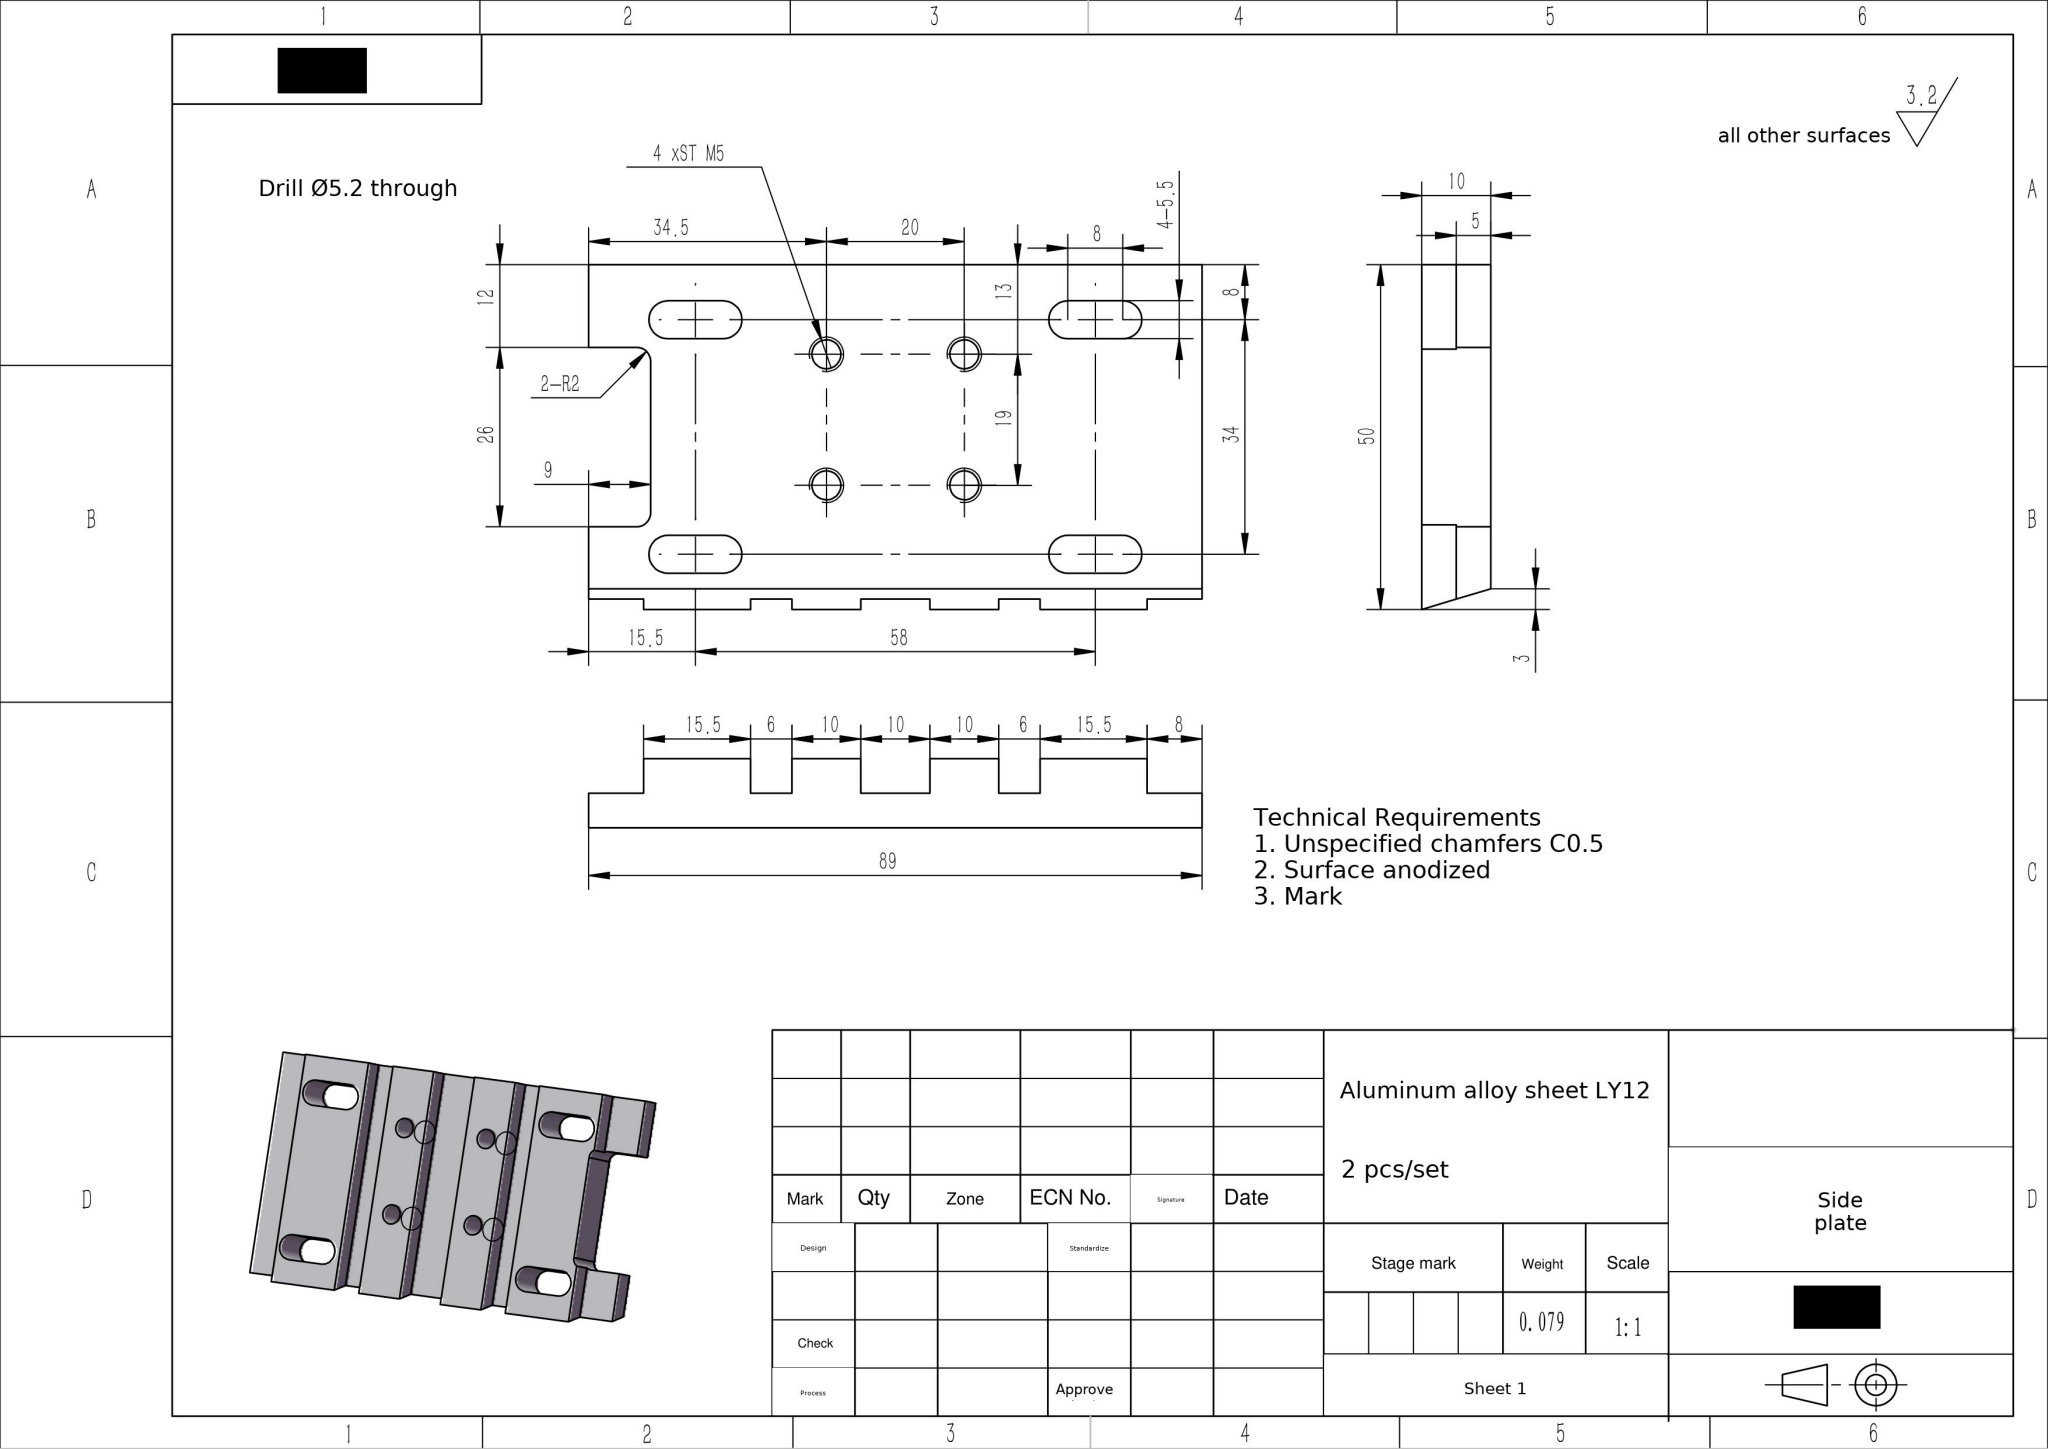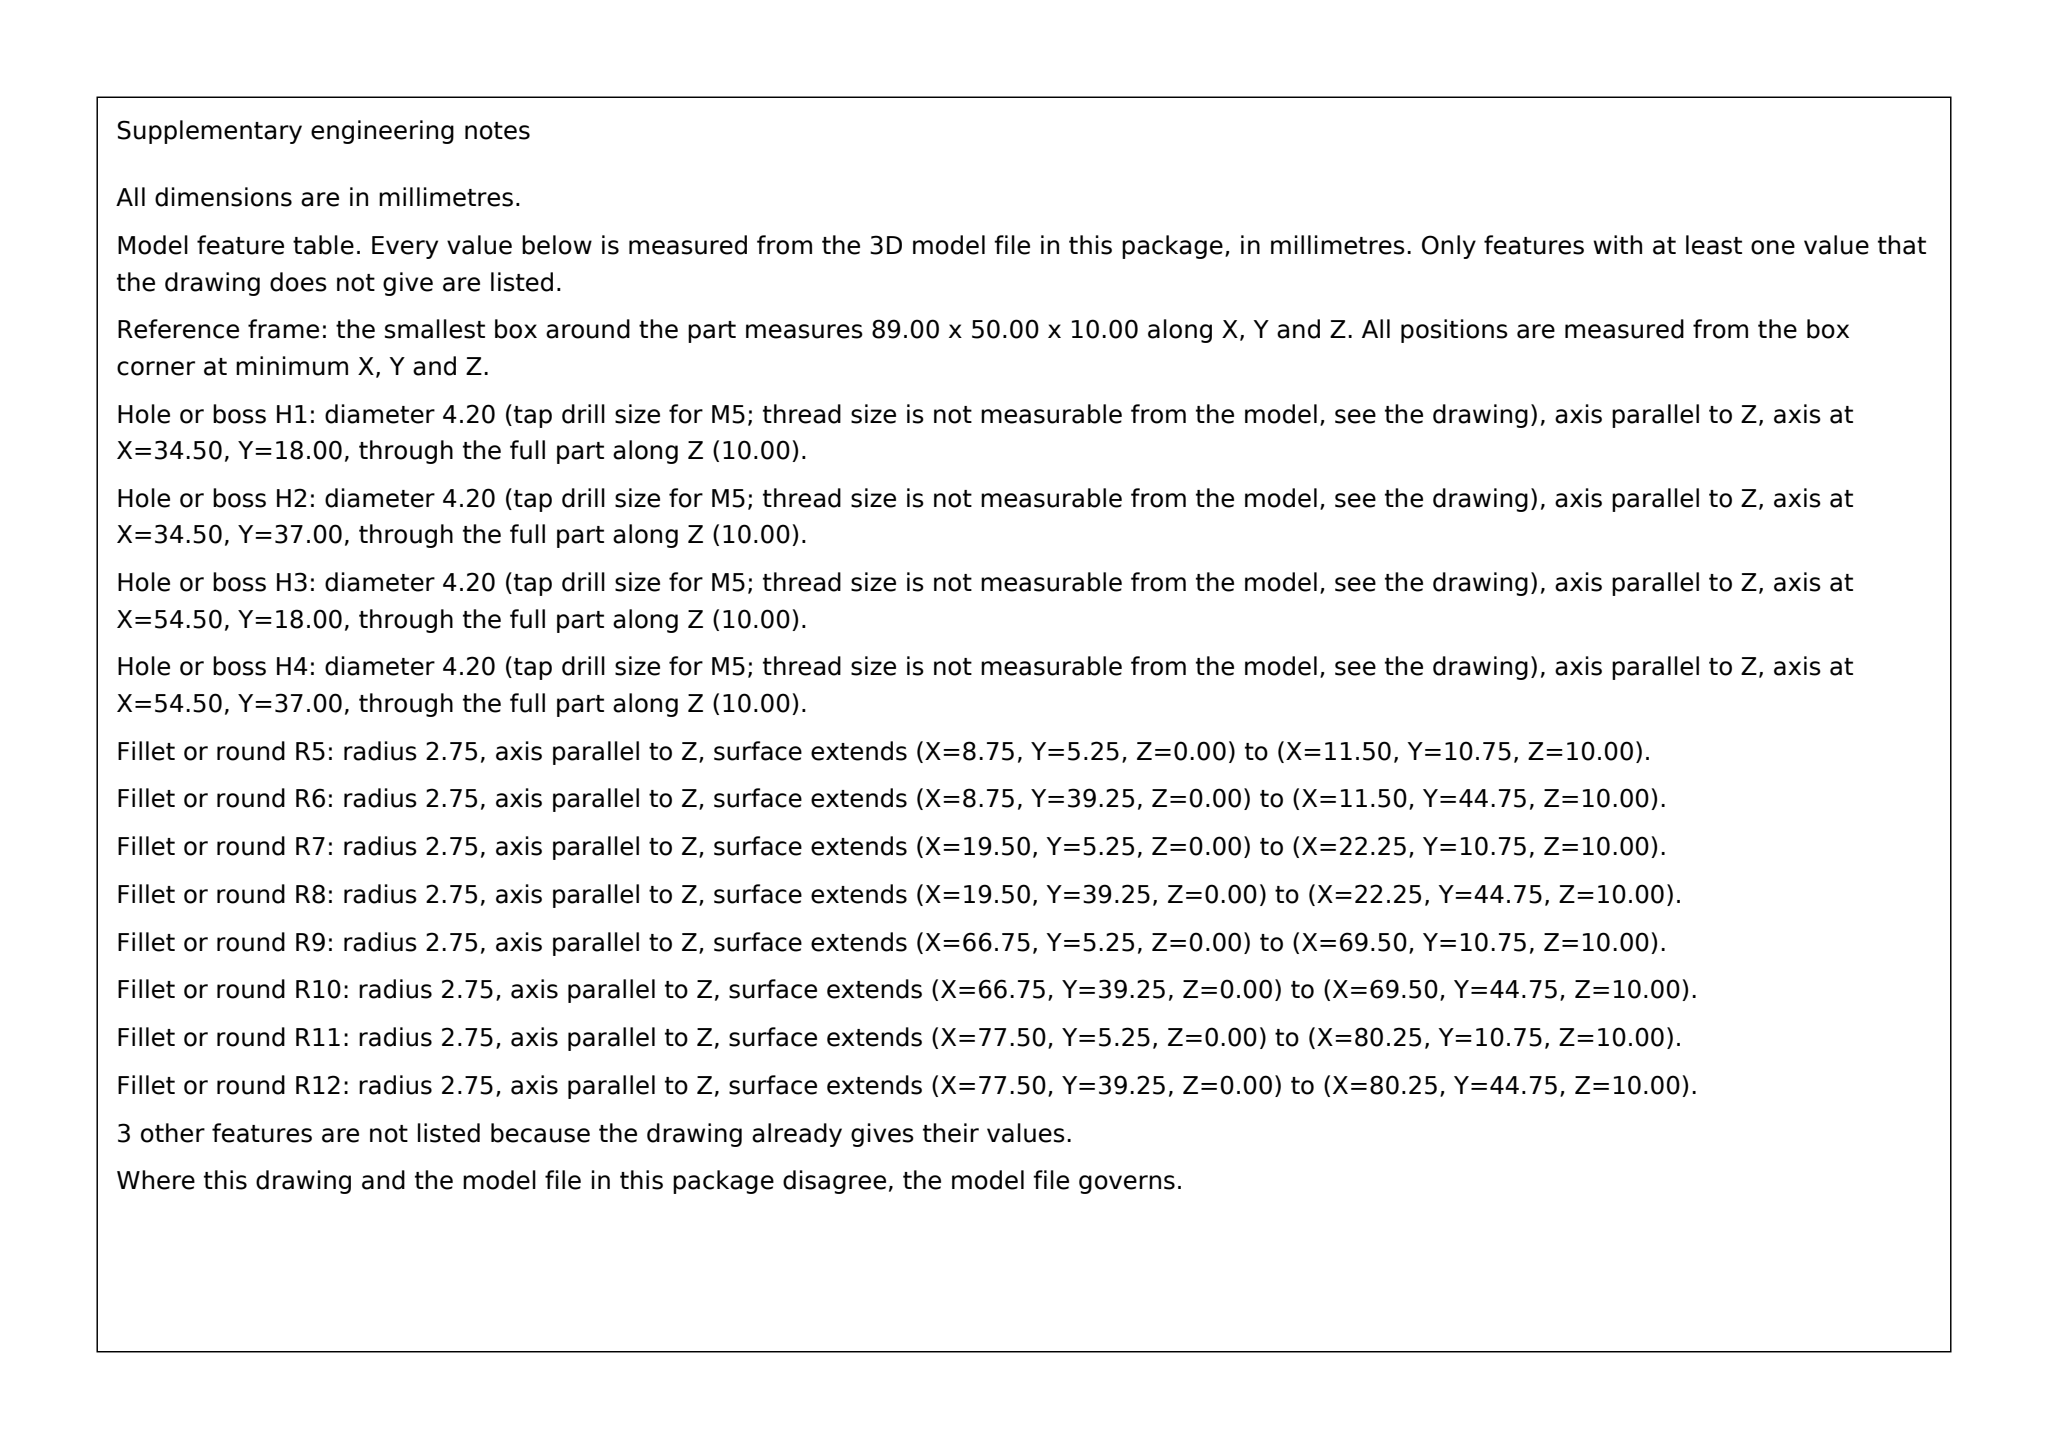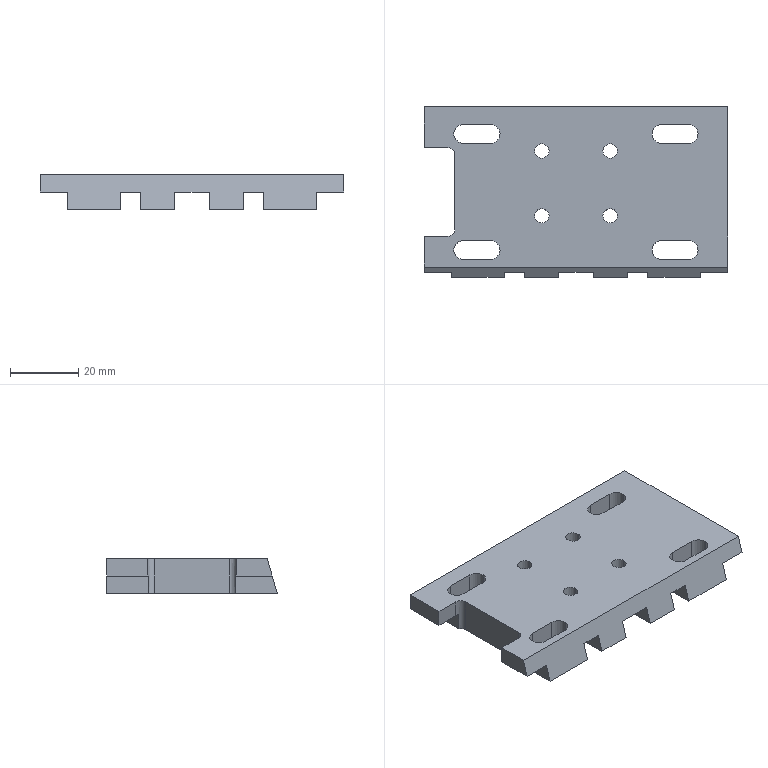Part | SolidWorks | mm | material Aluminum alloy sheet LY12 | 1 solid | 58 faces | box 89 x 50 x 10 mm | volume 29259 mm3 | plane 36 | cylinder 22 | commonest cylinder face diameters 5.5 x12 4.2 x8 4 x2